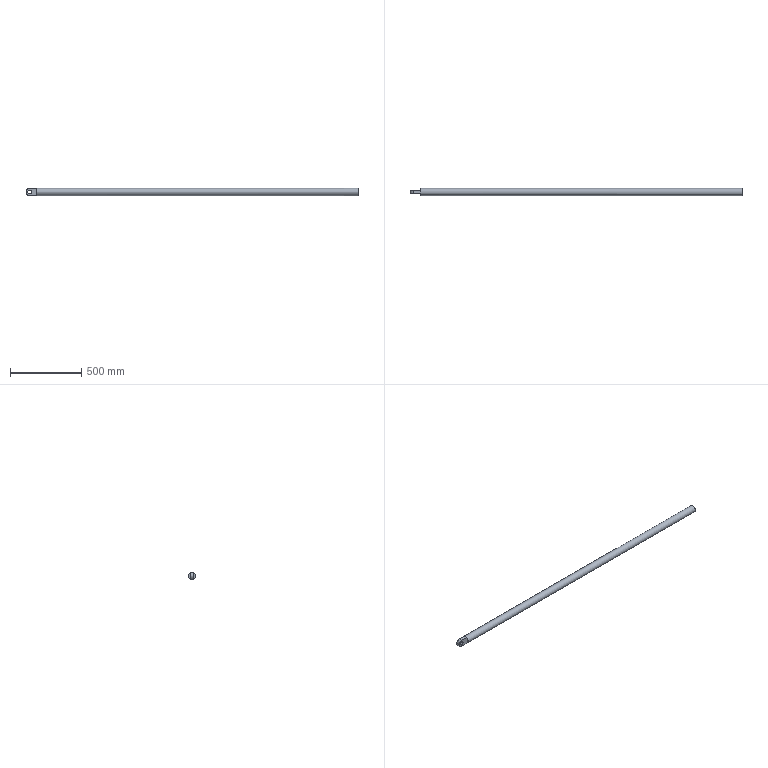Component | NX | SMALL_ARM_EXT_ROD | 1 solid | 14 faces | volume 4659054 mm3 | plane 11 | cylinder 3 | commonest cylinder face diameters 50.8 x2 25.4 x1